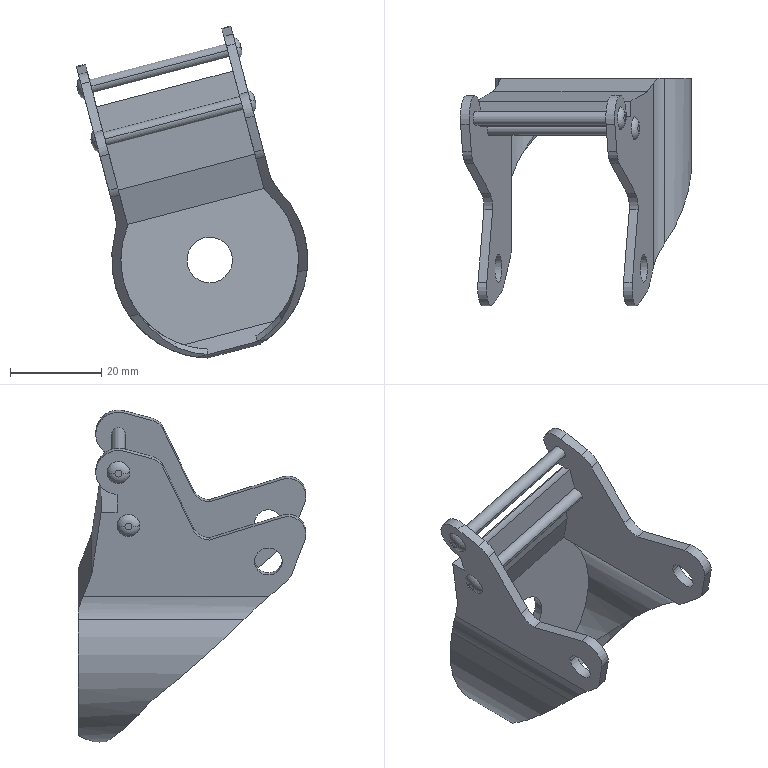Component | SolidWorks | PC-CAJ-P08-1_Rueda 2 in AZUL-1_Pieza3-1 | 1 solid | 75 faces | volume 11617 mm3 | plane 32 | cylinder 31 | torus 8 | spline 4 | commonest cylinder face diameters 8 x8 10 x7 3 x5 6.1 x4 39 x2 43 x2 20 x2 4 x1 | material Plain Carbon Steel